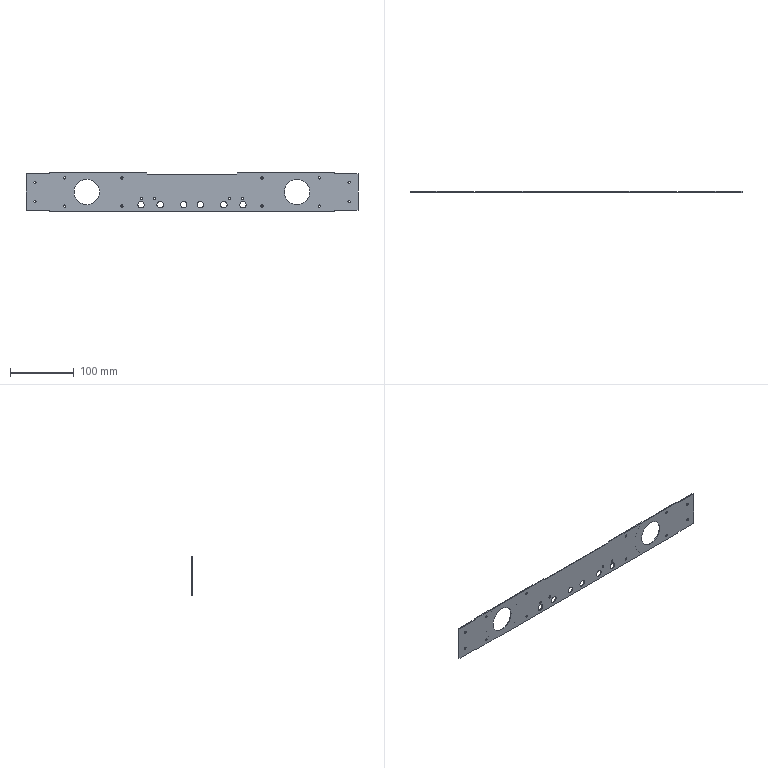CAM job | Mastercam | mm | 2 operations | part box 521 x 1.5 x 70
1. Contour (2D) | 10 - 10 平铣刀
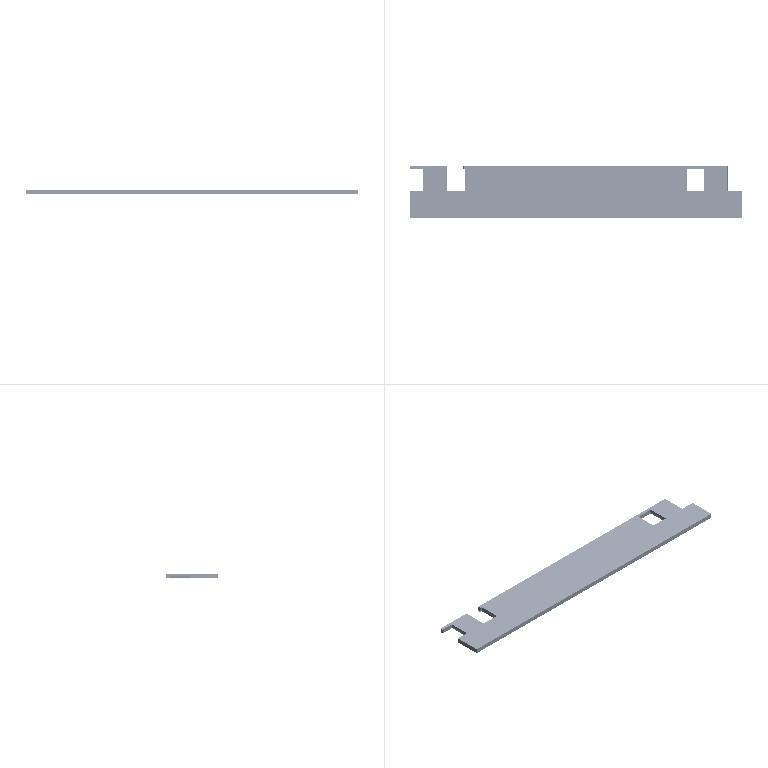2. Contour (2D) | 10 - 10 平铣刀